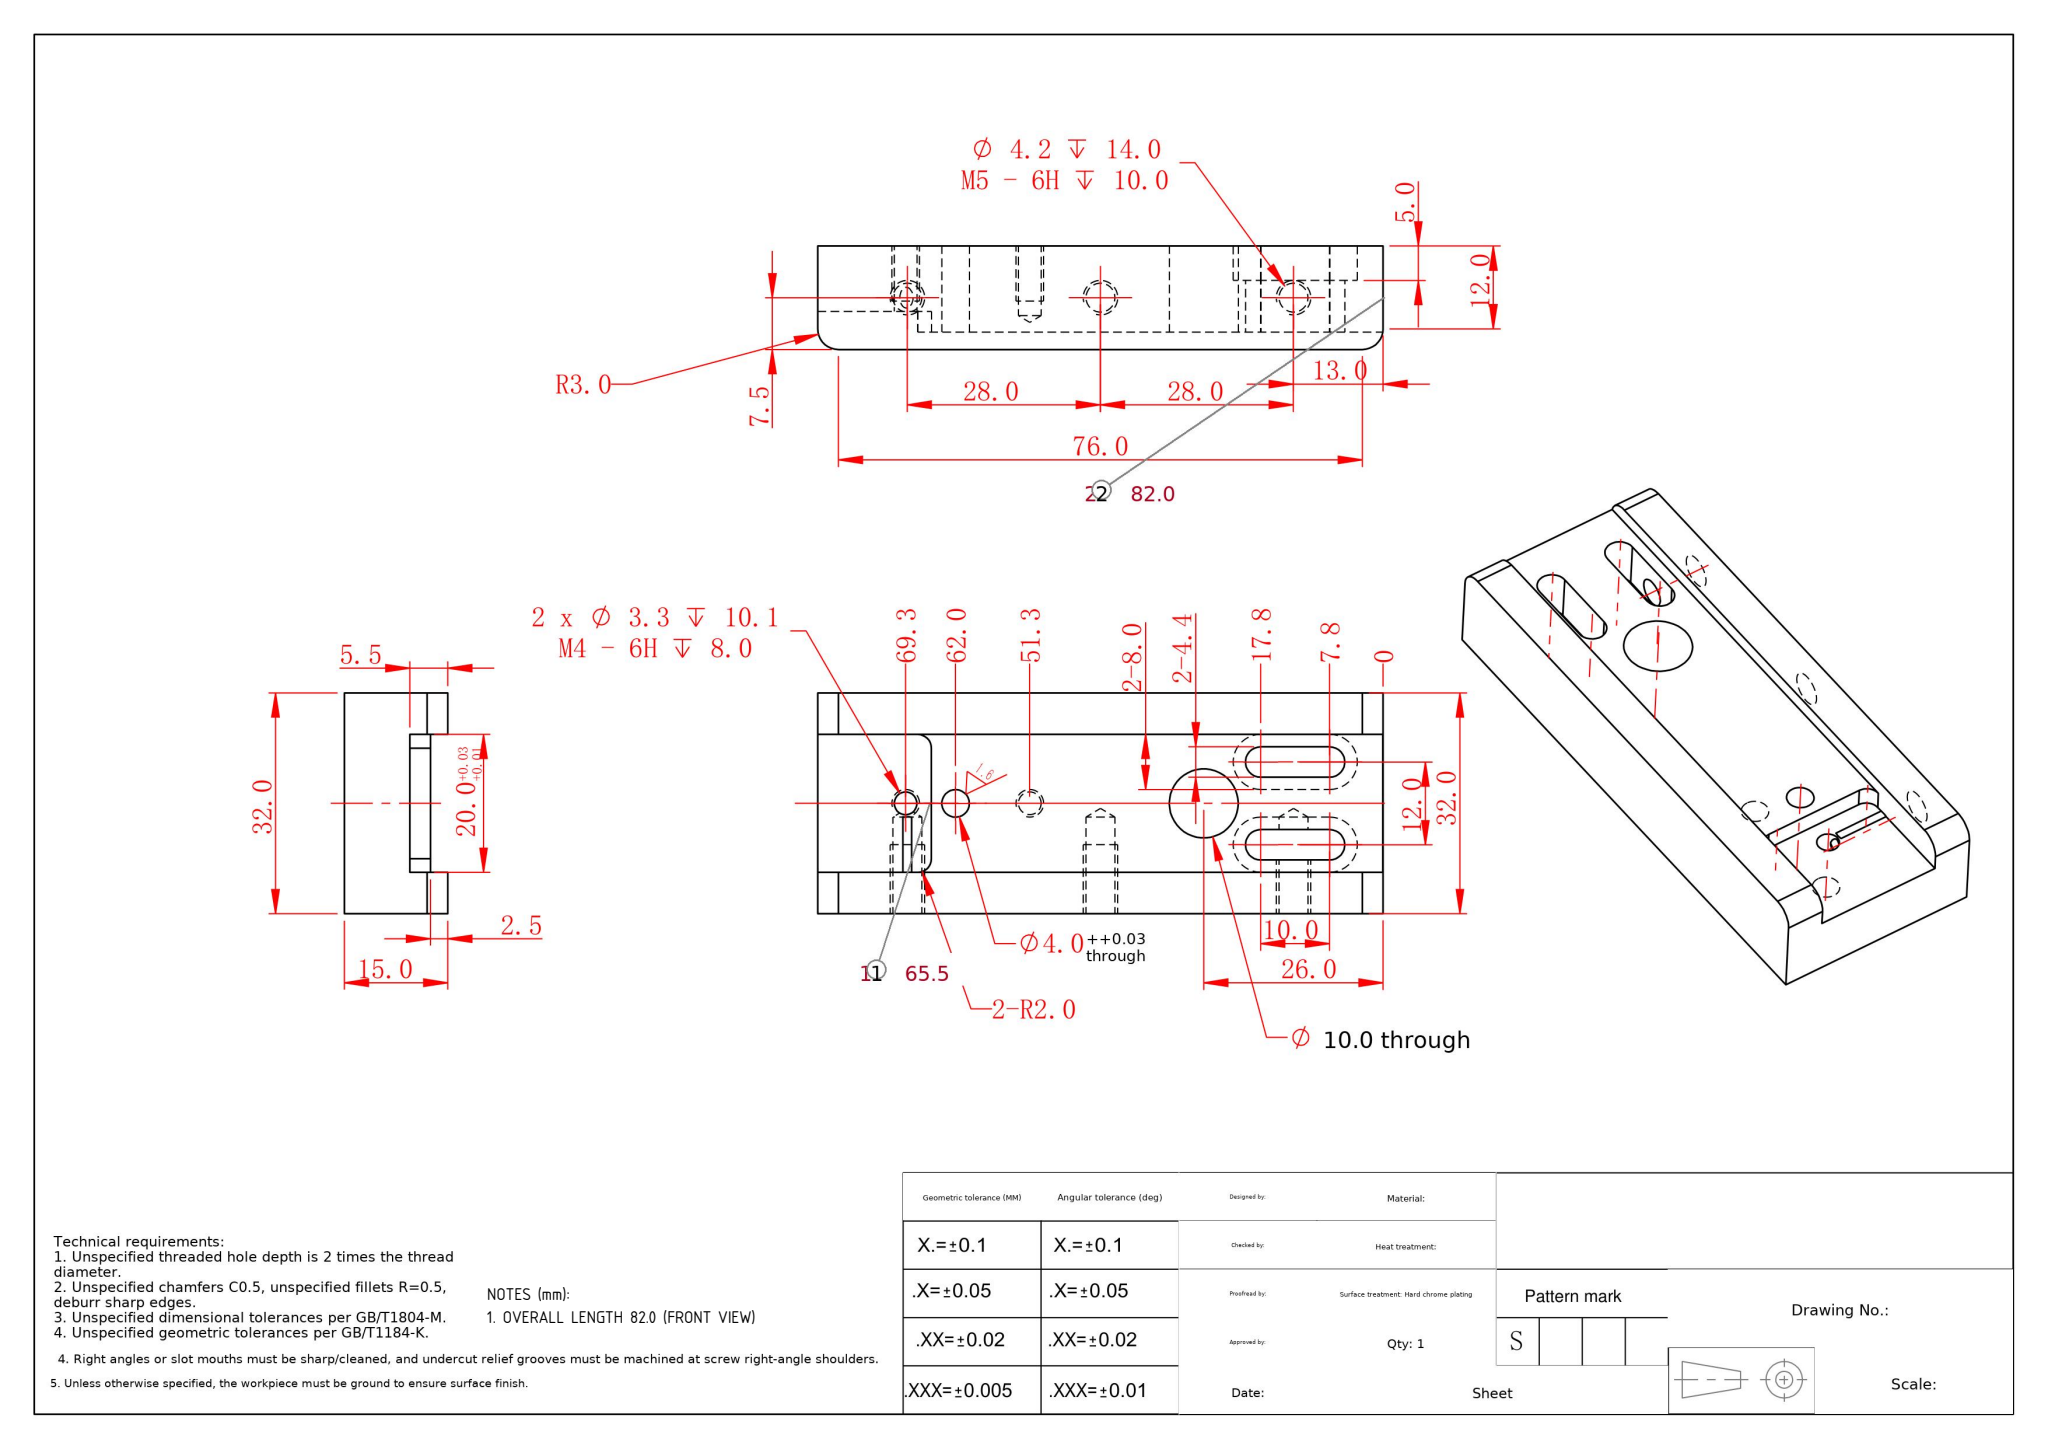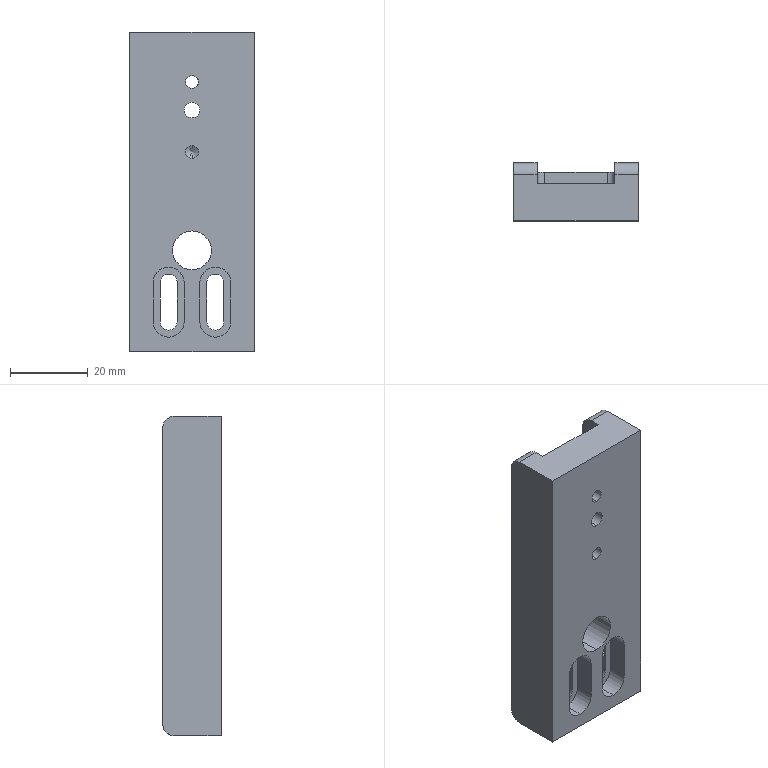Part | SolidWorks | mm | 1 solid | 63 faces | box 32 x 15 x 82 mm | volume 30192 mm3 | cylinder 33 | plane 22 | cone 8 | commonest cylinder face diameters 4.2 x8 8 x6 4.4 x6 3.3 x4 4 x4 6 x3 10 x2
Drawing notes:
OVERALL LENGTH 82.0 (FRONT VIEW) | from the solid: bbox_xyz z extent 0.0 to 82.0; faces z=0.0 and z=82.0
build123d program:
from build123d import *

# Parameters (mm, degrees)
SKETCH1_W             = 32
SKETCH1_H             = 82
BOSS_EXTRUDE1_DEPTH   = 15
SKETCH2_W             = 20
SKETCH2_H             = 2.5
CUT_EXTRUDE1_DEPTH    = 85.882
M5_TAPPED_HOLE1_D     = 4.2
M5_TAPPED_HOLE1_DEPTH = 14
M5_TAPPED_HOLE1_TIP   = 1.262
CUT_EXTRUDE2_REACH    = 48.497
SKETCH10_R            = 2
CUT_EXTRUDE3_DEPTH    = 3
M4_TAPPED_HOLE1_D     = 3.3
M4_TAPPED_HOLE1_DEPTH = 10.1
M4_TAPPED_HOLE1_TIP   = 0.9914
CUT_EXTRUDE4_REACH    = 48.497
CUT_EXTRUDE5_DEPTH    = 5
SKETCH16_R            = 5
CUT_EXTRUDE6_DEPTH    = 46.752
FILLET1_R             = 3


with BuildPart() as part:
    # Sketch1 → Boss-Extrude1 (new body)
    with BuildSketch(Plane(origin=(0, 0, 0), x_dir=(1, 0, 0), z_dir=(0, 1, 0))):
        Rectangle(SKETCH1_W, SKETCH1_H)
    extrude(amount=BOSS_EXTRUDE1_DEPTH)

    # Sketch2 → Cut-Extrude1 (cut, through all)
    with BuildSketch(Plane.XY.offset(41)):
        with Locations((0, 13.75)):
            Rectangle(SKETCH2_W, SKETCH2_H)
    extrude(amount=-CUT_EXTRUDE1_DEPTH, mode=Mode.SUBTRACT)

    # M5 Tapped Hole1
    with Locations(Plane(origin=(16, 0, 0), x_dir=(0, 0, 1), z_dir=(1, 0, 0))):
        with Locations((-28, -7.5), (0, -7.5), (28, -7.5)):
            Hole(M5_TAPPED_HOLE1_D / 2, depth=M5_TAPPED_HOLE1_DEPTH)
            with Locations((0, 0, -(M5_TAPPED_HOLE1_DEPTH + M5_TAPPED_HOLE1_TIP / 2))):  # 118° drill point
                Cone(0, M5_TAPPED_HOLE1_D / 2, M5_TAPPED_HOLE1_TIP, mode=Mode.SUBTRACT)

    # Sketch10 → Cut-Extrude2 (cut, up to next)
    with BuildSketch(Plane(origin=(0, 0, 0), x_dir=(-1, 0, 0), z_dir=(0, -1, 0)), mode=Mode.PRIVATE) as cut_extrude2_sk1:
        with Locations(Location((0, -21, 0), (0, 0, 90))):
            Circle(SKETCH10_R)
    cut_extrude2_tool1 = extrude(cut_extrude2_sk1.sketch, amount=-CUT_EXTRUDE2_REACH, mode=Mode.PRIVATE) & part.part
    add(cut_extrude2_tool1.solids().sort_by_distance((0, 0, 21))[0], mode=Mode.SUBTRACT)

    # Sketch11 → Cut-Extrude3 (cut)
    with BuildSketch(Plane(origin=(0, 12.5, 0), x_dir=(1, 0, 0), z_dir=(0, 1, 0))):
        with BuildLine():
            Line((10, -41), (-10, -41))
            Line((-10, -41), (-10, -26.5))
            ThreePointArc((-10, -26.5), (-9.414, -25.086), (-8, -24.5))
            Line((-8, -24.5), (8, -24.5))
            ThreePointArc((8, -24.5), (9.414, -25.086), (10, -26.5))
            Line((10, -26.5), (10, -41))
        make_face()
    extrude(amount=-CUT_EXTRUDE3_DEPTH, mode=Mode.SUBTRACT)

    # M4 Tapped Hole1
    with Locations(Plane(origin=(0, 0, 0), x_dir=(-1, 0, 0), z_dir=(0, -1, 0))):
        with Locations((0, -10.25), (0, -28.25)):
            Hole(M4_TAPPED_HOLE1_D / 2, depth=M4_TAPPED_HOLE1_DEPTH)
            with Locations((0, 0, -(M4_TAPPED_HOLE1_DEPTH + M4_TAPPED_HOLE1_TIP / 2))):  # 118° drill point
                Cone(0, M4_TAPPED_HOLE1_D / 2, M4_TAPPED_HOLE1_TIP, mode=Mode.SUBTRACT)

    # Sketch14 → Cut-Extrude4 (cut, up to next)
    with BuildSketch(Plane(origin=(0, 0, 0), x_dir=(-1, 0, 0), z_dir=(0, -1, 0)), mode=Mode.PRIVATE) as cut_extrude4_sk1:
        with BuildLine():
            Line((3.8, 23.25), (3.8, 33.25))
            ThreePointArc((3.8, 33.25), (6, 35.45), (8.2, 33.25))
            Line((8.2, 33.25), (8.2, 23.25))
            ThreePointArc((8.2, 23.25), (6, 21.05), (3.8, 23.25))
        make_face()
    cut_extrude4_tool1 = extrude(cut_extrude4_sk1.sketch, amount=-CUT_EXTRUDE4_REACH, mode=Mode.PRIVATE) & part.part
    # Sketch14 → Cut-Extrude4 (cut, up to next)
    with BuildSketch(Plane(origin=(0, 0, 0), x_dir=(-1, 0, 0), z_dir=(0, -1, 0)), mode=Mode.PRIVATE) as cut_extrude4_sk2:
        with BuildLine():
            Line((-8.2, 23.25), (-8.2, 33.25))
            ThreePointArc((-8.2, 33.25), (-6, 35.45), (-3.8, 33.25))
            Line((-3.8, 33.25), (-3.8, 23.25))
            ThreePointArc((-3.8, 23.25), (-6, 21.05), (-8.2, 23.25))
        make_face()
    cut_extrude4_tool2 = extrude(cut_extrude4_sk2.sketch, amount=-CUT_EXTRUDE4_REACH, mode=Mode.PRIVATE) & part.part
    add(cut_extrude4_tool1.solids().sort_by_distance((-6, 0, -28.25))[0], mode=Mode.SUBTRACT)
    add(cut_extrude4_tool2.solids().sort_by_distance((6, 0, -28.25))[0], mode=Mode.SUBTRACT)

    # Sketch15 → Cut-Extrude5 (cut)
    with BuildSketch(Plane.XZ):
        with BuildLine():
            Line((-2, -23.25), (-2, -33.25))
            ThreePointArc((-2, -33.25), (-6, -37.25), (-10, -33.25))
            Line((-10, -33.25), (-10, -23.25))
            ThreePointArc((-10, -23.25), (-6, -19.25), (-2, -23.25))
        make_face()
        with BuildLine():
            Line((10, -23.25), (10, -33.25))
            ThreePointArc((10, -33.25), (6, -37.25), (2, -33.25))
            Line((2, -33.25), (2, -23.25))
            ThreePointArc((2, -23.25), (6, -19.25), (10, -23.25))
        make_face()
    extrude(amount=-CUT_EXTRUDE5_DEPTH, mode=Mode.SUBTRACT)

    # Sketch16 → Cut-Extrude6 (cut, through all)
    with BuildSketch(Plane(origin=(0, 12.5, 0), x_dir=(1, 0, 0), z_dir=(0, 1, 0))):
        with Locations(Location((0, 15, 0), (0, 0, 270))):
            Circle(SKETCH16_R)
    extrude(amount=-CUT_EXTRUDE6_DEPTH, mode=Mode.SUBTRACT)

    # Fillet1
    fillet1_edges = [part.edges().sort_by_distance(p)[0] for p in [
        (13, 15, 41),
        (13, 15, -41),
        (-13, 15, 41),
    ]]
    fillet(fillet1_edges, radius=FILLET1_R)


solid = part.part